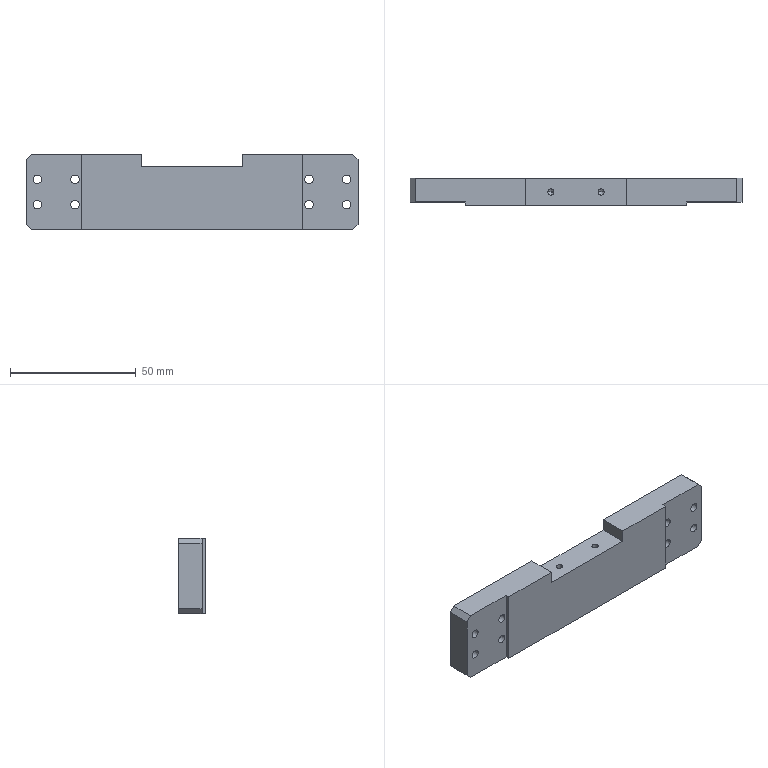Component | SolidWorks | SAWH02-03108A0MountingPlate8-2 | 1 solid | 112 faces | box 132 x 11 x 30 mm | volume 35349 mm3 | cylinder 60 | plane 28 | cone 24 | commonest cylinder face diameters 2.5 x24 6.5 x16 3.4 x16 8.2 x4 | material A6061
build123d program:
from build123d import *

# Parameters (mm, degrees)
SKETCH1_W                                       = 30
SKETCH1_H                                       = 132
BOSS_EXTRUDE1_DEPTH                             = 9.5
SKETCH13_W                                      = 30
SKETCH13_H                                      = 88
BOSS_EXTRUDE3_DEPTH                             = 1.5
M3_HEX_SOCKET_HEAD_CAP_SCREW_CBORE1_D           = 3.4
M3_HEX_SOCKET_HEAD_CAP_SCREW_CBORE1_CBORE_D     = 6.5
M3_HEX_SOCKET_HEAD_CAP_SCREW_CBORE1_CBORE_DEPTH = 3.4
M3_TAPPED_HOLE4_D                               = 2.5
M3_TAPPED_HOLE4_DEPTH                           = 8.5
M3_TAPPED_HOLE4_TIP                             = 0.7511
CHAMFER1_SIZE                                   = 2
SKETCH10_R                                      = 4.1
CUT_EXTRUDE3_DEPTH                              = 20
M3_TAPPED_HOLE2_D                               = 2.5
M3_TAPPED_HOLE2_DEPTH                           = 7.5
M3_TAPPED_HOLE2_TIP                             = 0.7511
SKETCH16_W                                      = 5
SKETCH16_H                                      = 40.2
CUT_EXTRUDE4_DEPTH                              = 69.571
M3_TAPPED_HOLE3_D                               = 2.5
M3_TAPPED_HOLE3_DEPTH                           = 7.5
M3_TAPPED_HOLE3_TIP                             = 0.7511


with BuildPart() as part:
    # Sketch1 → Boss-Extrude1 (new body)
    with BuildSketch(Plane(origin=(0, 0, 0), x_dir=(1, 0, 0), z_dir=(0, 1, 0))):
        Rectangle(SKETCH1_W, SKETCH1_H)
    extrude(amount=BOSS_EXTRUDE1_DEPTH)

    # Sketch13 → Boss-Extrude3 (add)
    with BuildSketch(Plane(origin=(0, 0, 0), x_dir=(-1, 0, 0), z_dir=(0, -1, 0))):
        Rectangle(SKETCH13_W, SKETCH13_H)
    extrude(amount=BOSS_EXTRUDE3_DEPTH)

    # M3 Hex Socket Head Cap Screw CBORE1 (through all)
    with Locations(Plane(origin=(0, 9.5, 0), x_dir=(1, 0, 0), z_dir=(0, 1, 0))):
        with Locations((-5, 46.5), (5, 46.5), (5, -46.5), (-5, -46.5), (-5, 61.5), (5, 61.5), (5, -61.5), (-5, -61.5)):
            CounterBoreHole(M3_HEX_SOCKET_HEAD_CAP_SCREW_CBORE1_D / 2, M3_HEX_SOCKET_HEAD_CAP_SCREW_CBORE1_CBORE_D / 2, M3_HEX_SOCKET_HEAD_CAP_SCREW_CBORE1_CBORE_DEPTH)

    # M3 Tapped Hole4
    with Locations(Plane(origin=(0, 9.5, 0), x_dir=(1, 0, 0), z_dir=(0, 1, 0))):
        with Locations((3, 35), (3, -35), (-5, 35), (-5, -35), (11, -35), (11, 35)):
            Hole(M3_TAPPED_HOLE4_D / 2, depth=M3_TAPPED_HOLE4_DEPTH)
            with Locations((0, 0, -(M3_TAPPED_HOLE4_DEPTH + M3_TAPPED_HOLE4_TIP / 2))):  # 118° drill point
                Cone(0, M3_TAPPED_HOLE4_D / 2, M3_TAPPED_HOLE4_TIP, mode=Mode.SUBTRACT)

    # Chamfer1
    chamfer1_edges = [part.edges().sort_by_distance(p)[0] for p in [
        (15, 4.75, 66),
        (-15, 4.75, 66),
        (-15, 4.75, -66),
        (15, 4.75, -66),
    ]]
    chamfer(chamfer1_edges, length=CHAMFER1_SIZE)

    # Sketch10 → Cut-Extrude3 (cut)
    with BuildSketch(Plane(origin=(15, 0, 0), x_dir=(0, 0, -1), z_dir=(1, 0, 0))):
        with Locations((-54, 5)):
            Circle(SKETCH10_R)
        with Locations((54, 5)):
            Circle(SKETCH10_R)
    extrude(amount=-CUT_EXTRUDE3_DEPTH, mode=Mode.SUBTRACT)

    # M3 Tapped Hole2
    with Locations(Plane(origin=(0, 9.5, 0), x_dir=(-1, 0, 0), z_dir=(0, 1, 0))):
        with Locations((-3.5, 10), (-11.5, 10), (-3.5, -10), (-11.5, -10)):
            Hole(M3_TAPPED_HOLE2_D / 2, depth=M3_TAPPED_HOLE2_DEPTH)
            with Locations((0, 0, -(M3_TAPPED_HOLE2_DEPTH + M3_TAPPED_HOLE2_TIP / 2))):  # 118° drill point
                Cone(0, M3_TAPPED_HOLE2_D / 2, M3_TAPPED_HOLE2_TIP, mode=Mode.SUBTRACT)

    # Sketch16 → Cut-Extrude4 (cut, through all)
    with BuildSketch(Plane(origin=(0, 9.5, 0), x_dir=(1, 0, 0), z_dir=(0, 1, 0))):
        with Locations((-12.5, 0)):
            Rectangle(SKETCH16_W, SKETCH16_H)
    extrude(amount=-CUT_EXTRUDE4_DEPTH, mode=Mode.SUBTRACT)

    # M3 Tapped Hole3
    with Locations(Plane.ZY.offset(10)):
        with Locations((-10, 4), (10, 4)):
            Hole(M3_TAPPED_HOLE3_D / 2, depth=M3_TAPPED_HOLE3_DEPTH)
            with Locations((0, 0, -(M3_TAPPED_HOLE3_DEPTH + M3_TAPPED_HOLE3_TIP / 2))):  # 118° drill point
                Cone(0, M3_TAPPED_HOLE3_D / 2, M3_TAPPED_HOLE3_TIP, mode=Mode.SUBTRACT)


solid = part.part

# Placed as in the assembly
solid = solid.moved(Location((27.51, -10.388, -110.792), (0, 90, 0)))